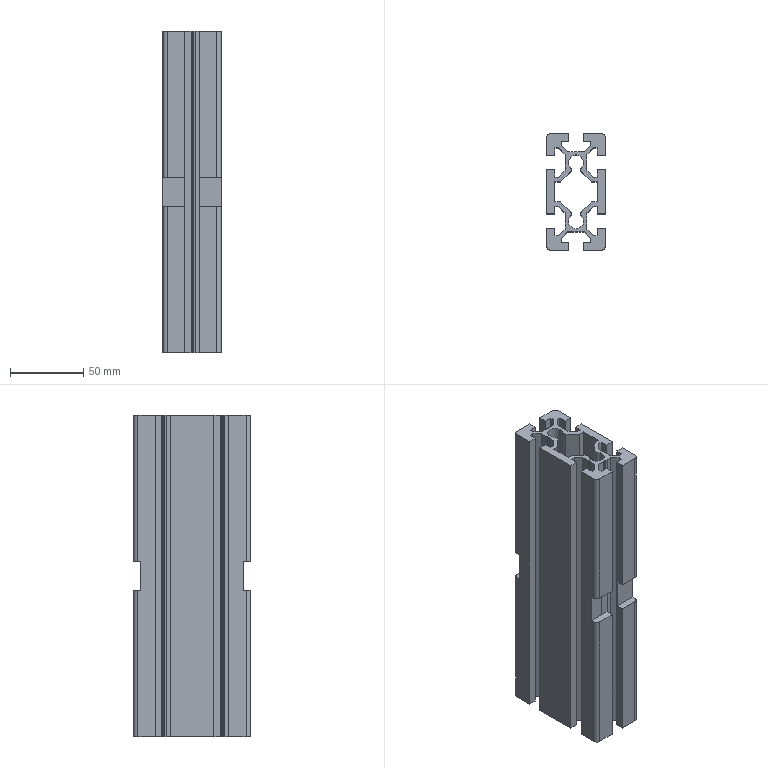Component | SolidWorks | Q1-A12-S21-Q1B.SLDASQ-1_Q1-GNFS8-4080-220-1 | 1 solid | 150 faces | box 40 x 80 x 220 mm | volume 288481 mm3 | plane 122 | cylinder 28 | commonest cylinder face diameters 1 x13 6 x8 4 x4 10.5 x3 | material 6061
build123d program:
from build123d import *

# Parameters (mm, degrees)
MISUMI_ALUMINUM_EXTRUSION_GNFS8_4080_1_DEPTH = 220
SKETCH12_W                                   = 20
SKETCH12_H                                   = 5
CUT_EXTRUDE1_DEPTH                           = 228.156


with BuildPart() as part:
    # Sketch11 → Misumi-Aluminum Extrusion GNFS8-4080_1 (new body)
    with BuildSketch(Plane.YZ):
        with BuildLine():
            Line((-17, -40), (-5, -40))
            Line((-5, -40), (-5, -34.5))
            Line((-5, -34.5), (-10, -34.5))
            Line((-10, -34.5), (-10, -31.768))
            Line((-10, -31.768), (-5.732, -27.5))
            Line((-5.732, -27.5), (-0.6536, -27.5))
            ThreePointArc((-0.6536, -27.5), (-0.5242, -27.483), (-0.4036, -27.433))
            Line((-0.4036, -27.433), (0, -27.2))
            Line((0, -27.2), (0.4036, -27.433))
            ThreePointArc((0.4036, -27.433), (0.6536, -27.5), (0.9036, -27.433))
            Line((0.9036, -27.433), (1.219, -27.251))
            Line((1.219, -27.251), (2.5, -27.5))
            Line((2.5, -27.5), (5.732, -27.5))
            Line((5.732, -27.5), (10, -31.768))
            Line((10, -31.768), (10, -34.5))
            Line((10, -34.5), (5, -34.5))
            Line((5, -34.5), (5, -40))
            Line((5, -40), (17, -40))
            ThreePointArc((17, -40), (19.121, -39.121), (20, -37))
            Line((20, -37), (20, -25))
            Line((20, -25), (14.5, -25))
            Line((14.5, -25), (14.5, -30))
            Line((14.5, -30), (11.768, -30))
            Line((11.768, -30), (7.5, -25.732))
            Line((7.5, -25.732), (7.5, -20.654))
            ThreePointArc((7.5, -20.654), (7.483, -20.524), (7.433, -20.404))
            Line((7.433, -20.404), (7.2, -20))
            Line((7.2, -20), (7.433, -19.596))
            ThreePointArc((7.433, -19.596), (7.5, -19.346), (7.433, -19.096))
            Line((7.433, -19.096), (7.251, -18.781))
            Line((7.251, -18.781), (7.5, -17.5))
            Line((7.5, -17.5), (7.5, -14.268))
            Line((7.5, -14.268), (11.768, -10))
            Line((11.768, -10), (14.5, -10))
            Line((14.5, -10), (14.5, -15))
            Line((14.5, -15), (20, -15))
            Line((20, -15), (20, 15))
            Line((20, 15), (14.5, 15))
            Line((14.5, 15), (14.5, 10))
            Line((14.5, 10), (11.768, 10))
            Line((11.768, 10), (7.5, 14.268))
            Line((7.5, 14.268), (7.5, 19.346))
            ThreePointArc((7.5, 19.346), (7.483, 19.476), (7.433, 19.596))
            Line((7.433, 19.596), (7.2, 20))
            Line((7.2, 20), (7.433, 20.404))
            ThreePointArc((7.433, 20.404), (7.5, 20.654), (7.433, 20.904))
            Line((7.433, 20.904), (7.251, 21.219))
            Line((7.251, 21.219), (7.5, 22.5))
            Line((7.5, 22.5), (7.5, 25.732))
            Line((7.5, 25.732), (11.768, 30))
            Line((11.768, 30), (14.5, 30))
            Line((14.5, 30), (14.5, 25))
            Line((14.5, 25), (20, 25))
            Line((20, 25), (20, 37))
            ThreePointArc((20, 37), (19.121, 39.121), (17, 40))
            Line((17, 40), (5, 40))
            Line((5, 40), (5, 34.5))
            Line((5, 34.5), (10, 34.5))
            Line((10, 34.5), (10, 31.768))
            Line((10, 31.768), (5.732, 27.5))
            Line((5.732, 27.5), (0.6536, 27.5))
            ThreePointArc((0.6536, 27.5), (0.5242, 27.483), (0.4036, 27.433))
            Line((0.4036, 27.433), (0, 27.2))
            Line((0, 27.2), (-0.4036, 27.433))
            ThreePointArc((-0.4036, 27.433), (-0.6536, 27.5), (-0.9036, 27.433))
            Line((-0.9036, 27.433), (-1.219, 27.251))
            Line((-1.219, 27.251), (-2.5, 27.5))
            Line((-2.5, 27.5), (-5.732, 27.5))
            Line((-5.732, 27.5), (-10, 31.768))
            Line((-10, 31.768), (-10, 34.5))
            Line((-10, 34.5), (-5, 34.5))
            Line((-5, 34.5), (-5, 40))
            Line((-5, 40), (-17, 40))
            ThreePointArc((-17, 40), (-19.121, 39.121), (-20, 37))
            Line((-20, 37), (-20, 25))
            Line((-20, 25), (-14.5, 25))
            Line((-14.5, 25), (-14.5, 30))
            Line((-14.5, 30), (-11.768, 30))
            Line((-11.768, 30), (-7.5, 25.732))
            Line((-7.5, 25.732), (-7.5, 20.654))
            ThreePointArc((-7.5, 20.654), (-7.483, 20.524), (-7.433, 20.404))
            Line((-7.433, 20.404), (-7.2, 20))
            Line((-7.2, 20), (-7.433, 19.596))
            ThreePointArc((-7.433, 19.596), (-7.5, 19.346), (-7.433, 19.096))
            Line((-7.433, 19.096), (-7.251, 18.781))
            Line((-7.251, 18.781), (-7.5, 17.5))
            Line((-7.5, 17.5), (-7.5, 14.268))
            Line((-7.5, 14.268), (-11.768, 10))
            Line((-11.768, 10), (-14.5, 10))
            Line((-14.5, 10), (-14.5, 15))
            Line((-14.5, 15), (-20, 15))
            Line((-20, 15), (-20, -15))
            Line((-20, -15), (-14.5, -15))
            Line((-14.5, -15), (-14.5, -10))
            Line((-14.5, -10), (-11.768, -10))
            Line((-11.768, -10), (-7.5, -14.268))
            Line((-7.5, -14.268), (-7.5, -19.346))
            ThreePointArc((-7.5, -19.346), (-7.483, -19.476), (-7.433, -19.596))
            Line((-7.433, -19.596), (-7.2, -20))
            Line((-7.2, -20), (-7.433, -20.404))
            ThreePointArc((-7.433, -20.404), (-7.5, -20.654), (-7.433, -20.904))
            Line((-7.433, -20.904), (-7.251, -21.219))
            Line((-7.251, -21.219), (-7.5, -22.5))
            Line((-7.5, -22.5), (-7.5, -25.732))
            Line((-7.5, -25.732), (-11.768, -30))
            Line((-11.768, -30), (-14.5, -30))
            Line((-14.5, -30), (-14.5, -25))
            Line((-14.5, -25), (-20, -25))
            Line((-20, -25), (-20, -37))
            ThreePointArc((-20, -37), (-19.121, -39.121), (-17, -40))
        make_face()
        with BuildLine():
            Line((-14.5, 7), (-14.5, -7))
            Line((-14.5, -7), (-10.525, -7))
            Line((-10.525, -7), (-3.886, -13.639))
            ThreePointArc((-3.886, -13.639), (-3.301, -15.019), (-3.838, -16.418))
            ThreePointArc((-3.838, -16.418), (0, -25.25), (3.838, -16.418))
            ThreePointArc((3.838, -16.418), (3.301, -15.019), (3.886, -13.639))
            Line((3.886, -13.639), (10.525, -7))
            Line((10.525, -7), (14.5, -7))
            Line((14.5, -7), (14.5, 7))
            Line((14.5, 7), (10.525, 7))
            Line((10.525, 7), (3.886, 13.639))
            ThreePointArc((3.886, 13.639), (3.301, 15.019), (3.838, 16.418))
            ThreePointArc((3.838, 16.418), (0, 25.25), (-3.838, 16.418))
            ThreePointArc((-3.838, 16.418), (-3.301, 15.019), (-3.886, 13.639))
            Line((-3.886, 13.639), (-10.525, 7))
            Line((-10.525, 7), (-14.5, 7))
        make_face(mode=Mode.SUBTRACT)
    extrude(amount=MISUMI_ALUMINUM_EXTRUSION_GNFS8_4080_1_DEPTH)

    # Sketch12 → Cut-Extrude1 (cut, through all)
    with BuildSketch(Plane(origin=(0, 20, 0), x_dir=(1, 0, 0), z_dir=(0, 1, 0))):
        with Locations((110, 37.5)):
            Rectangle(SKETCH12_W, SKETCH12_H)
        with Locations((110, -37.5)):
            Rectangle(SKETCH12_W, SKETCH12_H)
    extrude(amount=-CUT_EXTRUDE1_DEPTH, mode=Mode.SUBTRACT)


solid = part.part

# Placed as in the assembly
solid = solid.moved(Location((1738.5, 0, -110), (90, 0, 90)))